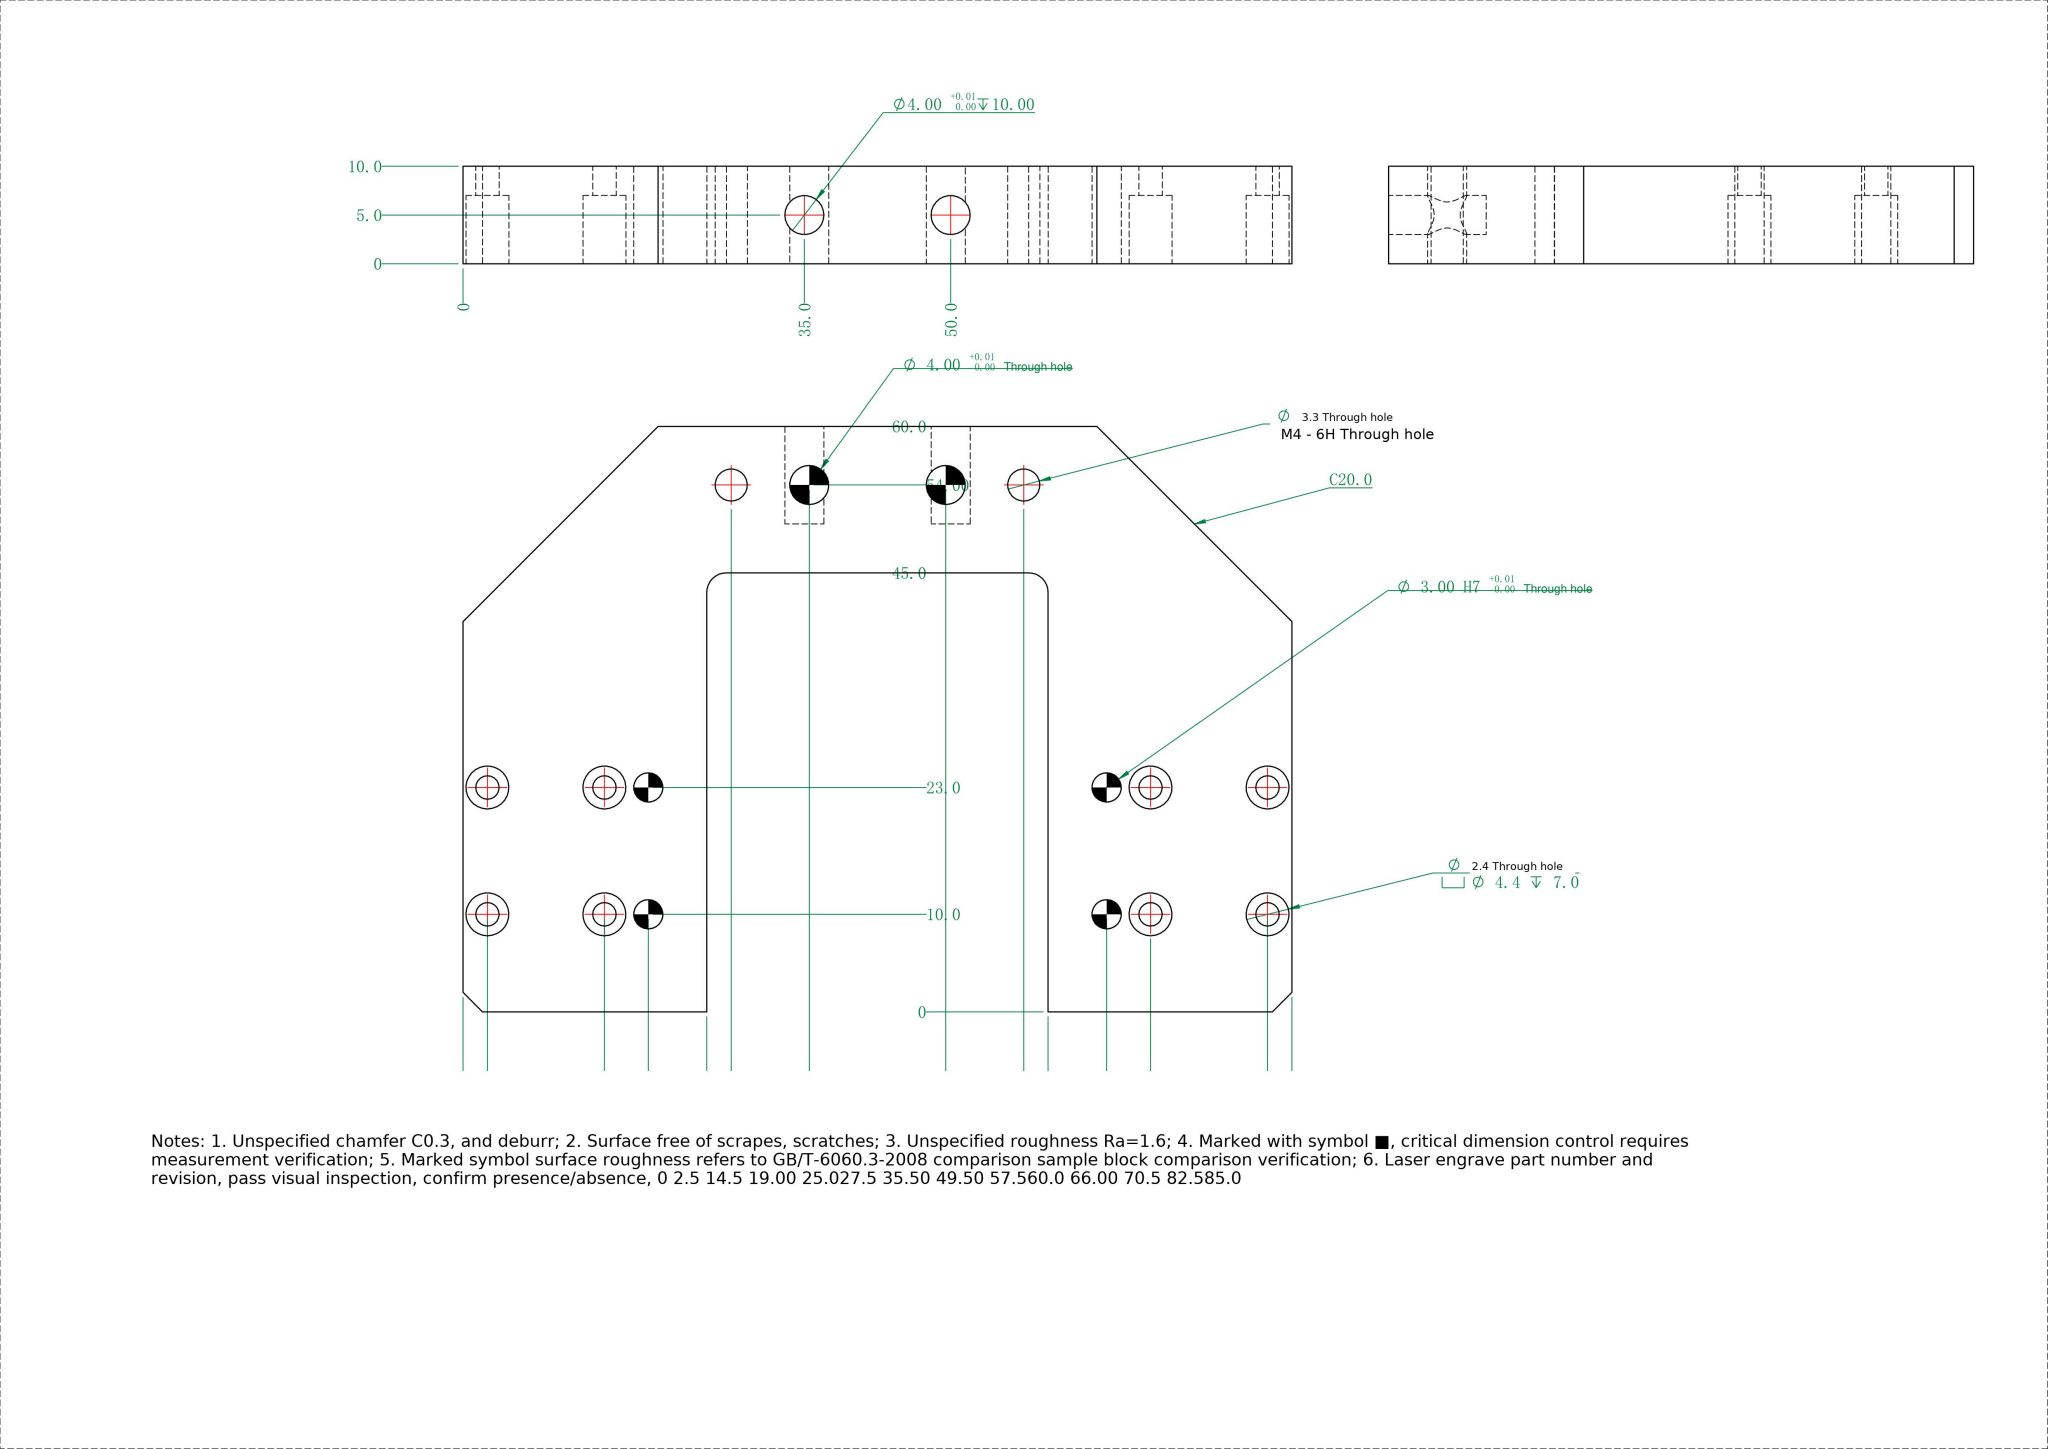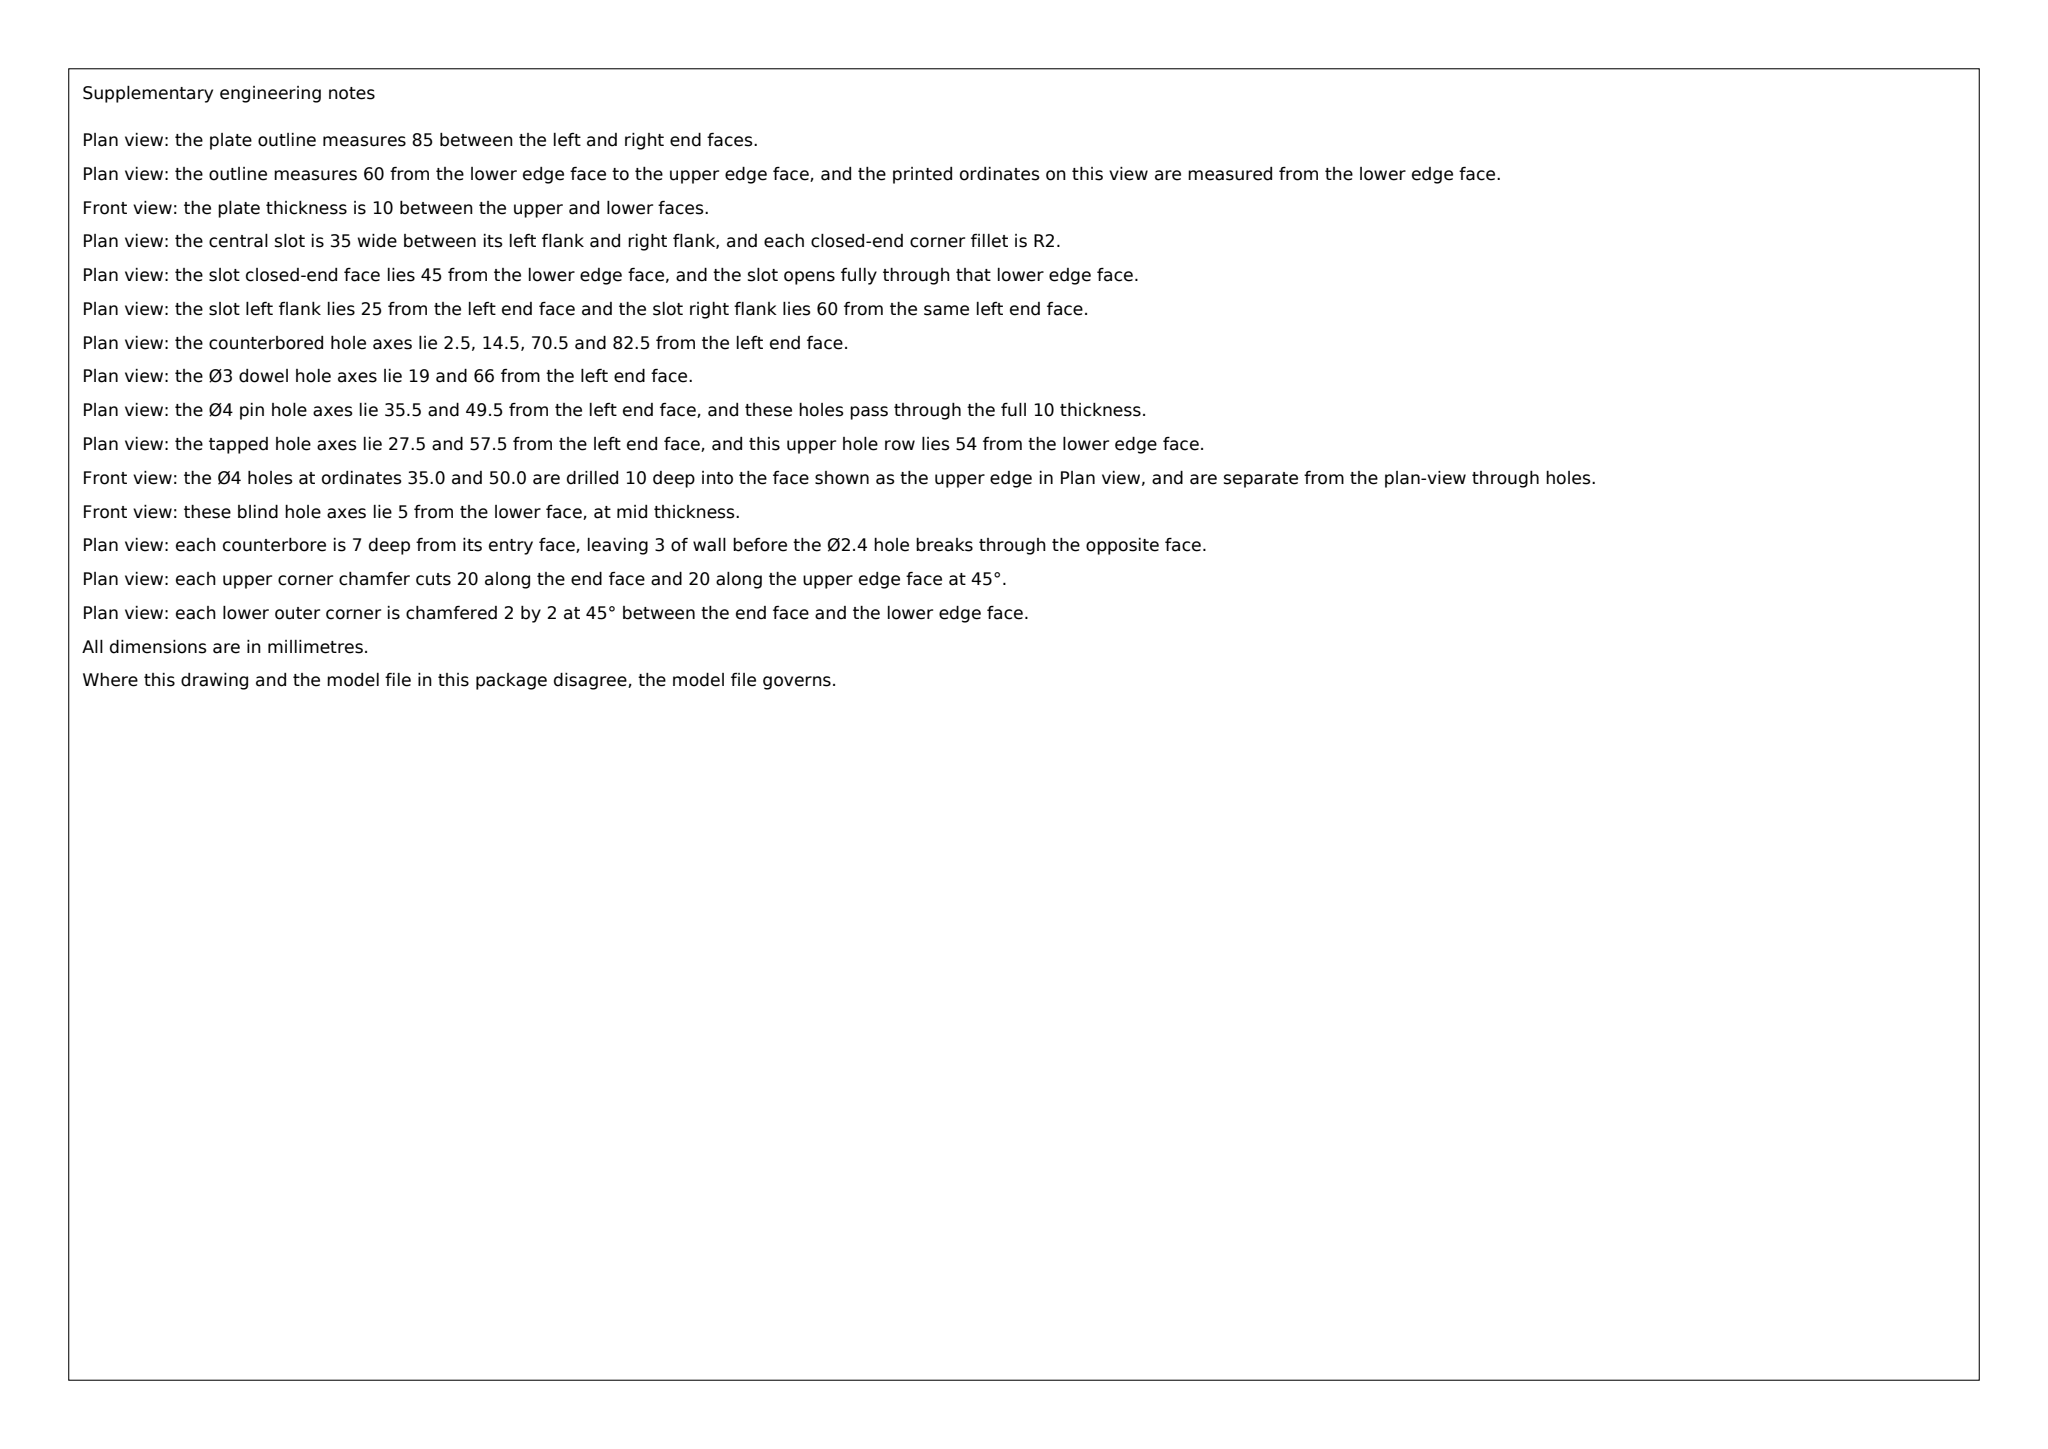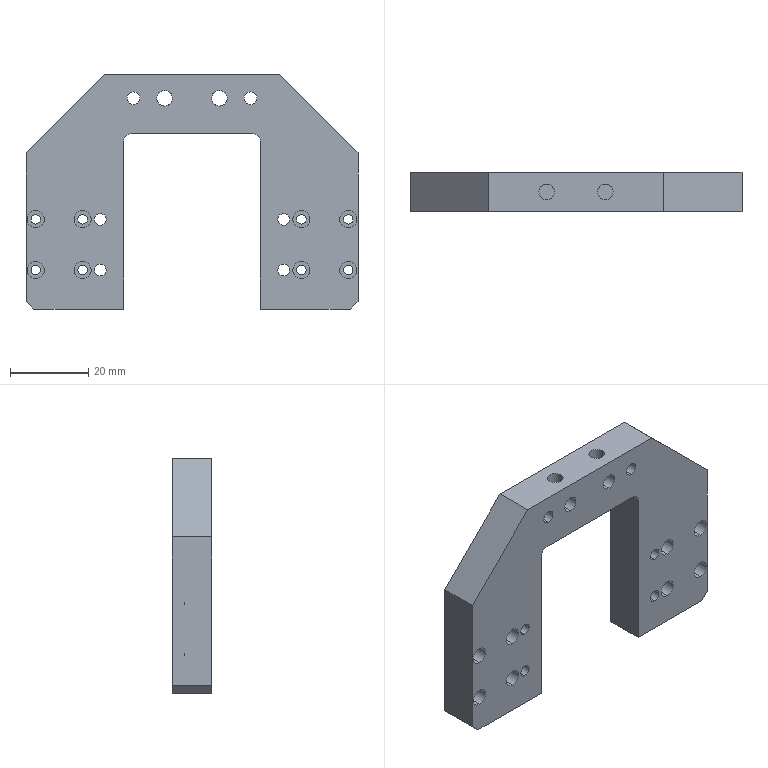Part | SolidWorks | mm | 1 solid | 80 faces | box 85 x 10 x 60 mm | volume 29390 mm3 | cylinder 56 | plane 24 | commonest cylinder face diameters 4.4 x16 2.4 x16 4 x12 3 x8 3.3 x4
Drawing notes:
OVERALL 85.0 W x 60.0 H x 10.0 THK; LH EDGE = X0 DATUM | from the solid: bbox_xyz [85.0,10.0,60.0]; planes x=0 and x=85
2X Ø3.3 M4-6H THRU AT Z54.0, X27.5 & X57.5 FROM LH EDGE | from the solid: Ø3.3 y-axis cyls at (27.5,54.0) & (57.5,54.0), length 10 thru
2X Ø4.00 THRU AT Z54.0, X35.5 & X49.5 FROM LH EDGE | from the solid: Ø4.0 y-axis cyls at (35.5,54.0) & (49.5,54.0), length 10 thru
2X Ø4.00 THRU AT Z43.0, X27.0 & X58.0 FROM LH EDGE | from the solid: Ø4.0 y-axis cyls at (27.0,43.0) & (58.0,43.0), length 10
4X Ø3.00 H7 THRU: X19.0 & X66.0 AT Z10.0 & Z23.0 | from the solid: Ø3.0 y-axis cyls at x=19.0 & 66.0, z=10.0 & 23.0, length 10
8X Ø2.4 THRU / Ø4.4 CBORE DP7.0: X2.5, 14.5, 70.5, 82.5 AT Z10.0 & Z23.0 | from the solid: Ø2.4 & Ø4.4 y-axis cyls at x=2.5,14.5,70.5,82.5, z=10.0 & 23.0
2X C20.0 TOP CORNERS, SYM ABT CL; TOP EDGE 45.0 WIDE | from the solid: Top face z=60 spans x=20..65 (45.0 wide) between side planes x=0 and x=85; equal 20x20 corner cuts both ends of 85.0 width
FRONT VIEW: CTR SLOT 35 WIDE X 45 HIGH, THRU FULL 10 THK | from the solid: x-planes 25.0 & 60.0 (35 apart) span z0-45 with z=45 ceiling plane; only y-faces are 0 and 10 (plus 7.0 c'bore floors), so region is through the full 10 thk, 2X z=0 leg bottoms
build123d program:
from build123d import *

# Parameters (mm, degrees)
SKETCH1_W                                       = 85
SKETCH1_H                                       = 75
BOSS_EXTRUDE1_DEPTH                             = 10
M4_TAPPED_HOLE1_D                               = 3.3
SIZE_MM_DOWEL_PIN_HOLE1_D                       = 4
M2_HEX_SOCKET_HEAD_CAP_SCREW_CBORE1_D           = 2.4
M2_HEX_SOCKET_HEAD_CAP_SCREW_CBORE1_CBORE_D     = 4.4
M2_HEX_SOCKET_HEAD_CAP_SCREW_CBORE1_CBORE_DEPTH = 7
SIZE_MM_DOWEL_PIN_HOLE1_2_D                     = 3
CHAMFER1_SIZE                                   = 2
CHAMFER3_SIZE                                   = 20
SKETCH14_W                                      = 85
SKETCH14_H                                      = 15
CUT_EXTRUDE1_DEPTH                              = 67.38
CUT_EXTRUDE2_DEPTH                              = 67.38
SKETCH16_R                                      = 2
CUT_EXTRUDE3_DEPTH                              = 10
CHAMFER4_SIZE                                   = 2
SKETCH17_W                                      = 35
SKETCH17_H                                      = 12
CUT_EXTRUDE4_DEPTH                              = 10


with BuildPart() as part:
    # Sketch1 → Boss-Extrude1 (new body)
    with BuildSketch(Plane(origin=(0, 10, 0), x_dir=(1, 0, 0), z_dir=(0, 1, 0))):
        with Locations((0, -12.5)):
            Rectangle(SKETCH1_W, SKETCH1_H)
    extrude(amount=-BOSS_EXTRUDE1_DEPTH)

    # M4 Tapped Hole1 (through all)
    with Locations(Plane(origin=(0, 0, 0), x_dir=(-1, 0, 0), z_dir=(0, -1, 0))):
        with Locations((15, -44), (-15, -44)):
            Hole(M4_TAPPED_HOLE1_D / 2)

    # Size mm Dowel Pin Hole1 (through all)
    with Locations(Plane(origin=(0, 0, 0), x_dir=(-1, 0, 0), z_dir=(0, -1, 0))):
        with Locations((7, -44), (-7, -44)):
            Hole(SIZE_MM_DOWEL_PIN_HOLE1_D / 2)

    # M2 Hex Socket Head Cap Screw CBORE1 (through all)
    with Locations(Plane.XZ):
        with Locations((-28, 0), (-40, 0), (-40, 13), (-28, 13), (28, 0), (28, 13), (40, 13), (40, 0)):
            CounterBoreHole(M2_HEX_SOCKET_HEAD_CAP_SCREW_CBORE1_D / 2, M2_HEX_SOCKET_HEAD_CAP_SCREW_CBORE1_CBORE_D / 2, M2_HEX_SOCKET_HEAD_CAP_SCREW_CBORE1_CBORE_DEPTH)

    # Size mm Dowel Pin Hole1_2 (through all)
    with Locations(Plane(origin=(0, 10, 0), x_dir=(1, 0, 0), z_dir=(0, 1, 0))):
        with Locations((-23.5, 0), (-23.5, -13), (23.5, 0), (23.5, -13)):
            Hole(SIZE_MM_DOWEL_PIN_HOLE1_2_D / 2)

    # Chamfer1
    chamfer1_edges = [part.edges().sort_by_distance(p)[0] for p in [
        (42.5, 5, -25),
        (-42.5, 5, -25),
    ]]
    chamfer(chamfer1_edges, length=CHAMFER1_SIZE)

    # Chamfer3
    chamfer3_edges = [part.edges().sort_by_distance(p)[0] for p in [
        (42.5, 5, 50),
        (-42.5, 5, 50),
    ]]
    chamfer(chamfer3_edges, length=CHAMFER3_SIZE)

    # Sketch14 → Cut-Extrude1 (cut, through all)
    with BuildSketch(Plane(origin=(0, 0, 0), x_dir=(-1, 0, 0), z_dir=(0, -1, 0))):
        with Locations((0, 17.5)):
            Rectangle(SKETCH14_W, SKETCH14_H)
    extrude(amount=-CUT_EXTRUDE1_DEPTH, mode=Mode.SUBTRACT)

    # Sketch15 → Cut-Extrude2 (cut, through all)
    with BuildSketch(Plane(origin=(0, 0, 0), x_dir=(-1, 0, 0), z_dir=(0, -1, 0))):
        with BuildLine():
            Line((-15.5, 0), (15.5, 0))
            ThreePointArc((15.5, 0), (16.914, -0.5858), (17.5, -2))
            Line((17.5, -2), (17.5, -33))
            ThreePointArc((17.5, -33), (16.914, -34.414), (15.5, -35))
            Line((15.5, -35), (-15.5, -35))
            ThreePointArc((-15.5, -35), (-16.914, -34.414), (-17.5, -33))
            Line((-17.5, -33), (-17.5, -2))
            ThreePointArc((-17.5, -2), (-16.914, -0.5858), (-15.5, 0))
        make_face()
    extrude(amount=-CUT_EXTRUDE2_DEPTH, mode=Mode.SUBTRACT)

    # Sketch16 → Cut-Extrude3 (cut)
    with BuildSketch(Plane.XY.offset(50)):
        with Locations((-7.5, 5)):
            Circle(SKETCH16_R)
        with Locations((7.5, 5)):
            Circle(SKETCH16_R)
    extrude(amount=-CUT_EXTRUDE3_DEPTH, mode=Mode.SUBTRACT)

    # Chamfer4
    chamfer4_edges = [part.edges().sort_by_distance(p)[0] for p in [
        (42.5, 5, -10),
        (-42.5, 5, -10),
    ]]
    chamfer(chamfer4_edges, length=CHAMFER4_SIZE)

    # Sketch17 → Cut-Extrude4 (cut)
    with BuildSketch(Plane.XZ):
        with Locations((0, -4)):
            Rectangle(SKETCH17_W, SKETCH17_H)
    extrude(amount=-CUT_EXTRUDE4_DEPTH, mode=Mode.SUBTRACT)


solid = part.part